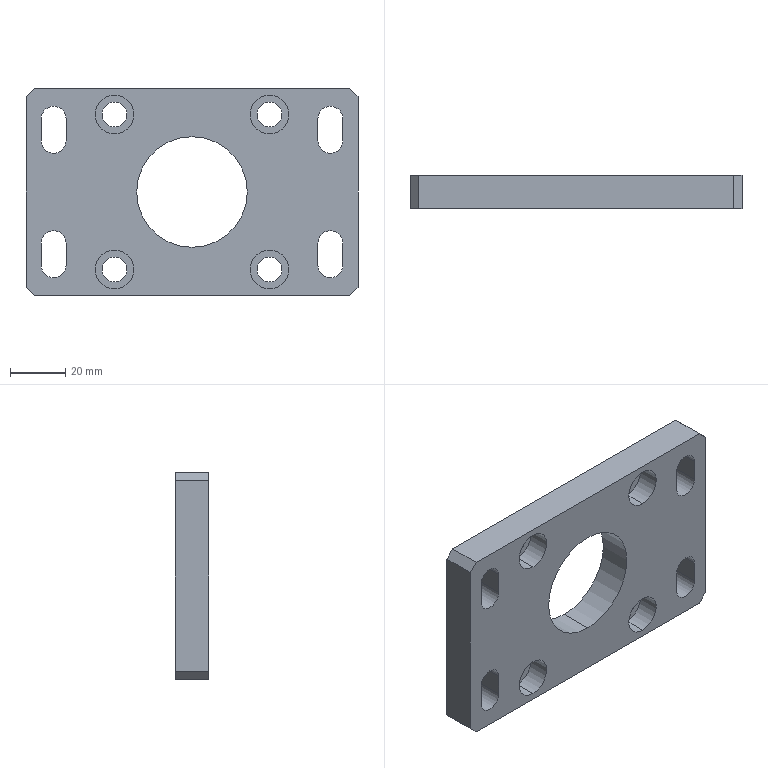Component | SolidWorks | -UpperPullCylinderMountingPlate-1 | 1 solid | 52 faces | box 120 x 12 x 75 mm | volume 80251 mm3 | cylinder 30 | plane 22 | commonest cylinder face diameters 9 x20 14 x8 40 x2
build123d program:
from build123d import *

# Parameters (mm, degrees)
SKETCH1_W                                           = 120
SKETCH1_H                                           = 75
BOSS_EXTRUDE1_DEPTH                                 = 6
CHAMFER1_SIZE                                       = 3
SKETCH2_R                                           = 20
CUT_EXTRUDE1_DEPTH                                  = 72.765
CYLINDRICAL_COUNTERSUNK_HOLE_FOR_M8_HEX_D           = 9
CYLINDRICAL_COUNTERSUNK_HOLE_FOR_M8_HEX_DEPTH       = 20
CYLINDRICAL_COUNTERSUNK_HOLE_FOR_M8_HEX_CBORE_D     = 14
CYLINDRICAL_COUNTERSUNK_HOLE_FOR_M8_HEX_CBORE_DEPTH = 8
CYLINDRICAL_COUNTERSUNK_HOLE_FOR_M8_HEX_TIP         = 2.704
CUT_EXTRUDE2_DEPTH                                  = 72.765


with BuildPart() as part:
    # Sketch1 → Boss-Extrude1 (new, symmetric)
    with BuildSketch(Plane(origin=(0, 0, 0), x_dir=(1, 0, 0), z_dir=(0, 1, 0))):
        Rectangle(SKETCH1_W, SKETCH1_H)
    extrude(amount=BOSS_EXTRUDE1_DEPTH, both=True)

    # Chamfer1
    chamfer1_edges = [part.edges().sort_by_distance(p)[0] for p in [
        (-60, 0, -37.5),
        (60, 0, -37.5),
        (60, 0, 37.5),
        (-60, 0, 37.5),
    ]]
    chamfer(chamfer1_edges, length=CHAMFER1_SIZE)

    # Sketch2 → Cut-Extrude1 (cut, through all)
    with BuildSketch(Plane(origin=(0, 6, 0), x_dir=(1, 0, 0), z_dir=(0, 1, 0))):
        with Locations(Location((0, 0, 0), (0, 0, 270))):
            Circle(SKETCH2_R)
    extrude(amount=-CUT_EXTRUDE1_DEPTH, mode=Mode.SUBTRACT)

    # Cylindrical Countersunk Hole for M8 Hex
    with Locations(Plane(origin=(0, -6, 0), x_dir=(-1, 0, 0), z_dir=(0, -1, 0))):
        with Locations((28, -28), (-28, -28), (-28, 28), (28, 28)):
            CounterBoreHole(CYLINDRICAL_COUNTERSUNK_HOLE_FOR_M8_HEX_D / 2, CYLINDRICAL_COUNTERSUNK_HOLE_FOR_M8_HEX_CBORE_D / 2, CYLINDRICAL_COUNTERSUNK_HOLE_FOR_M8_HEX_CBORE_DEPTH, depth=CYLINDRICAL_COUNTERSUNK_HOLE_FOR_M8_HEX_DEPTH)
            with Locations((0, 0, -(CYLINDRICAL_COUNTERSUNK_HOLE_FOR_M8_HEX_DEPTH + CYLINDRICAL_COUNTERSUNK_HOLE_FOR_M8_HEX_TIP / 2))):  # 118° drill point
                Cone(0, CYLINDRICAL_COUNTERSUNK_HOLE_FOR_M8_HEX_D / 2, CYLINDRICAL_COUNTERSUNK_HOLE_FOR_M8_HEX_TIP, mode=Mode.SUBTRACT)

    # Sketch5 → Cut-Extrude2 (cut, through all)
    with BuildSketch(Plane(origin=(0, 6, 0), x_dir=(1, 0, 0), z_dir=(0, 1, 0))):
        with BuildLine():
            Line((-45.5, 26.5), (-45.5, 18.5))
            ThreePointArc((-45.5, 18.5), (-50, 14), (-54.5, 18.5))
            Line((-54.5, 18.5), (-54.5, 26.5))
            ThreePointArc((-54.5, 26.5), (-50, 31), (-45.5, 26.5))
        make_face()
        with BuildLine():
            Line((54.5, 26.5), (54.5, 18.5))
            ThreePointArc((54.5, 18.5), (50, 14), (45.5, 18.5))
            Line((45.5, 18.5), (45.5, 26.5))
            ThreePointArc((45.5, 26.5), (50, 31), (54.5, 26.5))
        make_face()
    cut_extrude2 = extrude(amount=-CUT_EXTRUDE2_DEPTH, mode=Mode.SUBTRACT)

    # Mirror1: Cut-Extrude2 across plane
    add(cut_extrude2.mirror(Plane.XY), mode=Mode.SUBTRACT)


solid = part.part

# Placed as in the assembly
solid = solid.moved(Location((30, 1457, -120), (0, 0, 0)))